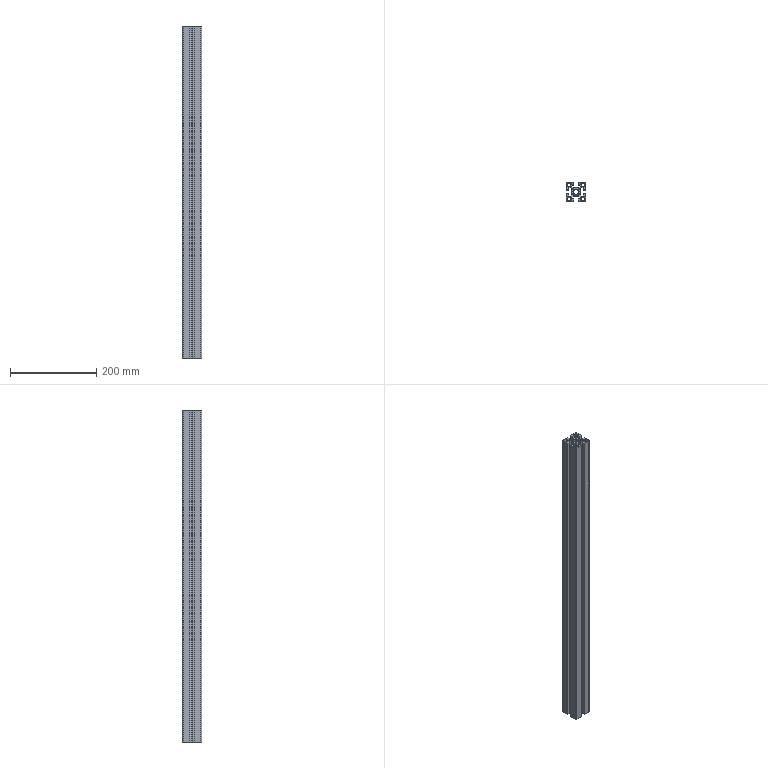Component | SolidWorks | HFS8_4545_04-B-1 | 1 solid | 131 faces | box 45 x 45 x 772 mm | volume 619299 mm3 | plane 82 | cylinder 49 | commonest cylinder face diameters 2 x18 3 x12 1 x10 12.5 x5 6 x4
build123d program:
from build123d import *

# Parameters (mm, degrees)
BOSS_EXTRUDE1_DEPTH = 772


with BuildPart() as part:
    # Sketch1 → Boss-Extrude1 (new body)
    with BuildSketch(Plane.XY):
        with BuildLine():
            Line((-19.5, -22.5), (-5, -22.5))
            Line((-5, -22.5), (-5, -16.5))
            Line((-5, -16.5), (-10, -16.5))
            Line((-10, -16.5), (-10, -13))
            Line((-10, -13), (-6.5, -9.5))
            Line((-6.5, -9.5), (-1.212, -9.5))
            Line((-1.212, -9.5), (0, -8.8))
            Line((0, -8.8), (1.212, -9.5))
            Line((1.212, -9.5), (6.5, -9.5))
            Line((6.5, -9.5), (10, -13))
            Line((10, -13), (10, -16.5))
            Line((10, -16.5), (5, -16.5))
            Line((5, -16.5), (5, -22.5))
            Line((5, -22.5), (19.5, -22.5))
            ThreePointArc((19.5, -22.5), (21.621, -21.621), (22.5, -19.5))
            Line((22.5, -19.5), (22.5, -5))
            Line((22.5, -5), (16.5, -5))
            Line((16.5, -5), (16.5, -10))
            Line((16.5, -10), (13, -10))
            Line((13, -10), (9.5, -6.5))
            Line((9.5, -6.5), (9.5, -1.212))
            Line((9.5, -1.212), (8.8, 0))
            Line((8.8, 0), (9.5, 1.212))
            Line((9.5, 1.212), (9.5, 6.5))
            Line((9.5, 6.5), (13, 10))
            Line((13, 10), (16.5, 10))
            Line((16.5, 10), (16.5, 5))
            Line((16.5, 5), (22.5, 5))
            Line((22.5, 5), (22.5, 19.5))
            ThreePointArc((22.5, 19.5), (21.621, 21.621), (19.5, 22.5))
            Line((19.5, 22.5), (5, 22.5))
            Line((5, 22.5), (5, 16.5))
            Line((5, 16.5), (10, 16.5))
            Line((10, 16.5), (10, 13))
            Line((10, 13), (6.5, 9.5))
            Line((6.5, 9.5), (1.212, 9.5))
            Line((1.212, 9.5), (0, 8.8))
            Line((0, 8.8), (-1.212, 9.5))
            Line((-1.212, 9.5), (-6.5, 9.5))
            Line((-6.5, 9.5), (-10, 13))
            Line((-10, 13), (-10, 16.5))
            Line((-10, 16.5), (-5, 16.5))
            Line((-5, 16.5), (-5, 22.5))
            Line((-5, 22.5), (-19.5, 22.5))
            ThreePointArc((-19.5, 22.5), (-21.621, 21.621), (-22.5, 19.5))
            Line((-22.5, 19.5), (-22.5, 5))
            Line((-22.5, 5), (-16.5, 5))
            Line((-16.5, 5), (-16.5, 10))
            Line((-16.5, 10), (-13, 10))
            Line((-13, 10), (-9.5, 6.5))
            Line((-9.5, 6.5), (-9.5, 1.212))
            Line((-9.5, 1.212), (-8.8, 0))
            Line((-8.8, 0), (-9.5, -1.212))
            Line((-9.5, -1.212), (-9.5, -6.5))
            Line((-9.5, -6.5), (-13, -10))
            Line((-13, -10), (-16.5, -10))
            Line((-16.5, -10), (-16.5, -5))
            Line((-16.5, -5), (-22.5, -5))
            Line((-22.5, -5), (-22.5, -19.5))
            ThreePointArc((-22.5, -19.5), (-21.621, -21.621), (-19.5, -22.5))
        make_face()
        with BuildLine():
            Line((12, 18.5), (12, 13))
            ThreePointArc((12, 13), (12.293, 12.293), (13, 12))
            Line((13, 12), (18.5, 12))
            ThreePointArc((18.5, 12), (19.5, 11), (20.5, 12))
            Line((20.5, 12), (20.5, 19.5))
            ThreePointArc((20.5, 19.5), (20.207, 20.207), (19.5, 20.5))
            Line((19.5, 20.5), (12, 20.5))
            ThreePointArc((12, 20.5), (11, 19.5), (12, 18.5))
        make_face(mode=Mode.SUBTRACT)
        with BuildLine():
            Line((12, -20.5), (19.5, -20.5))
            ThreePointArc((19.5, -20.5), (20.207, -20.207), (20.5, -19.5))
            Line((20.5, -19.5), (20.5, -12))
            ThreePointArc((20.5, -12), (19.5, -11), (18.5, -12))
            Line((18.5, -12), (13, -12))
            ThreePointArc((13, -12), (12.293, -12.293), (12, -13))
            Line((12, -13), (12, -18.5))
            ThreePointArc((12, -18.5), (11, -19.5), (12, -20.5))
        make_face(mode=Mode.SUBTRACT)
        with BuildLine():
            Line((-4.725, -6.139), (-3.947, -5.361))
            ThreePointArc((-3.947, -5.361), (-3.649, -5.217), (-3.327, -5.291))
            ThreePointArc((-3.327, -5.291), (0, -6.25), (3.327, -5.291))
            ThreePointArc((3.327, -5.291), (3.649, -5.217), (3.947, -5.361))
            Line((3.947, -5.361), (4.725, -6.139))
            ThreePointArc((4.725, -6.139), (7.283, -7.283), (6.139, -4.725))
            Line((6.139, -4.725), (5.361, -3.947))
            ThreePointArc((5.361, -3.947), (5.217, -3.649), (5.291, -3.327))
            ThreePointArc((5.291, -3.327), (6.25, 0), (5.291, 3.327))
            ThreePointArc((5.291, 3.327), (5.217, 3.649), (5.361, 3.947))
            Line((5.361, 3.947), (6.139, 4.725))
            ThreePointArc((6.139, 4.725), (7.283, 7.283), (4.725, 6.139))
            Line((4.725, 6.139), (3.947, 5.361))
            ThreePointArc((3.947, 5.361), (3.649, 5.217), (3.327, 5.291))
            ThreePointArc((3.327, 5.291), (0, 6.25), (-3.327, 5.291))
            ThreePointArc((-3.327, 5.291), (-3.649, 5.217), (-3.947, 5.361))
            Line((-3.947, 5.361), (-4.725, 6.139))
            ThreePointArc((-4.725, 6.139), (-7.283, 7.283), (-6.139, 4.725))
            Line((-6.139, 4.725), (-5.361, 3.947))
            ThreePointArc((-5.361, 3.947), (-5.217, 3.649), (-5.291, 3.327))
            ThreePointArc((-5.291, 3.327), (-6.25, 0), (-5.291, -3.327))
            ThreePointArc((-5.291, -3.327), (-5.217, -3.649), (-5.361, -3.947))
            Line((-5.361, -3.947), (-6.139, -4.725))
            ThreePointArc((-6.139, -4.725), (-7.283, -7.283), (-4.725, -6.139))
        make_face(mode=Mode.SUBTRACT)
        with BuildLine():
            Line((-19.5, -20.5), (-12, -20.5))
            ThreePointArc((-12, -20.5), (-11, -19.5), (-12, -18.5))
            Line((-12, -18.5), (-12, -13))
            ThreePointArc((-12, -13), (-12.293, -12.293), (-13, -12))
            Line((-13, -12), (-18.5, -12))
            ThreePointArc((-18.5, -12), (-19.5, -11), (-20.5, -12))
            Line((-20.5, -12), (-20.5, -19.5))
            ThreePointArc((-20.5, -19.5), (-20.207, -20.207), (-19.5, -20.5))
        make_face(mode=Mode.SUBTRACT)
        with BuildLine():
            Line((-18.5, 12), (-13, 12))
            ThreePointArc((-13, 12), (-12.293, 12.293), (-12, 13))
            Line((-12, 13), (-12, 18.5))
            ThreePointArc((-12, 18.5), (-11, 19.5), (-12, 20.5))
            Line((-12, 20.5), (-19.5, 20.5))
            ThreePointArc((-19.5, 20.5), (-20.207, 20.207), (-20.5, 19.5))
            Line((-20.5, 19.5), (-20.5, 12))
            ThreePointArc((-20.5, 12), (-19.5, 11), (-18.5, 12))
        make_face(mode=Mode.SUBTRACT)
    extrude(amount=-BOSS_EXTRUDE1_DEPTH)


solid = part.part

# Placed as in the assembly
solid = solid.moved(Location((-65.506, -746.913, -470.928), (0, 0, 0)))